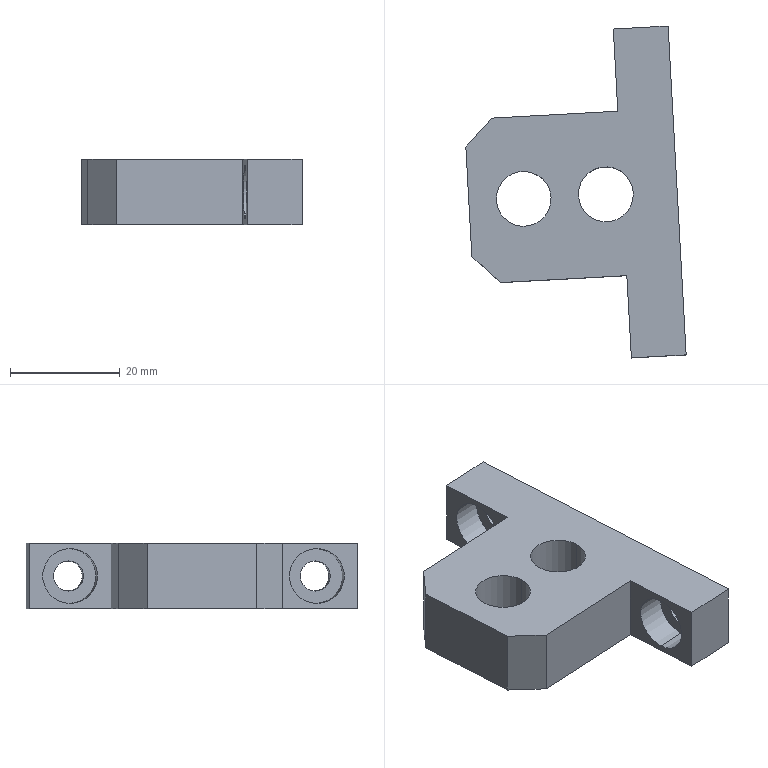Component | SolidWorks | BearingPressPartK-1 | 1 solid | 26 faces | box 40.13 x 60.46 x 12 mm | volume 14028 mm3 | plane 14 | cylinder 12 | commonest cylinder face diameters 10 x8 5.5 x4
build123d program:
from build123d import *

# Parameters (mm, degrees)
SKETCH1_W                                       = 38
SKETCH1_H                                       = 30
BOSS_EXTRUDE1_DEPTH                             = 12
M10X1_25_TAPPED_HOLE1_D                         = 10
M10X1_25_TAPPED_HOLE1_DEPTH                     = 23.75
M10X1_25_TAPPED_HOLE1_TIP                       = 3.004
CHAMFER1_SIZE                                   = 5
SKETCH6_W                                       = 10
SKETCH6_H                                       = 12
BOSS_EXTRUDE2_DEPTH                             = 15
SKETCH7_W                                       = 10
SKETCH7_H                                       = 12
BOSS_EXTRUDE3_DEPTH                             = 15
M5_HEX_SOCKET_HEAD_CAP_SCREW_CBORE1_D           = 5.5
M5_HEX_SOCKET_HEAD_CAP_SCREW_CBORE1_CBORE_D     = 10
M5_HEX_SOCKET_HEAD_CAP_SCREW_CBORE1_CBORE_DEPTH = 5.4


with BuildPart() as part:
    # Sketch1 → Boss-Extrude1 (new body)
    with BuildSketch(Plane.XY):
        with Locations((19, 15)):
            Rectangle(SKETCH1_W, SKETCH1_H)
    extrude(amount=BOSS_EXTRUDE1_DEPTH)

    # M10x1.25 Tapped Hole1
    with Locations(Plane.XY.offset(12)):
        with Locations((25, 15), (10, 15)):
            Hole(M10X1_25_TAPPED_HOLE1_D / 2, depth=M10X1_25_TAPPED_HOLE1_DEPTH)
            with Locations((0, 0, -(M10X1_25_TAPPED_HOLE1_DEPTH + M10X1_25_TAPPED_HOLE1_TIP / 2))):  # 118° drill point
                Cone(0, M10X1_25_TAPPED_HOLE1_D / 2, M10X1_25_TAPPED_HOLE1_TIP, mode=Mode.SUBTRACT)

    # Chamfer1
    chamfer1_edges = [part.edges().sort_by_distance(p)[0] for p in [
        (0, 30, 6),
        (0, 0, 6),
    ]]
    chamfer(chamfer1_edges, length=CHAMFER1_SIZE)

    # Sketch6 → Boss-Extrude2 (add)
    with BuildSketch(Plane.XZ):
        with Locations((33, 6)):
            Rectangle(SKETCH6_W, SKETCH6_H)
    extrude(amount=BOSS_EXTRUDE2_DEPTH)

    # Sketch7 → Boss-Extrude3 (add)
    with BuildSketch(Plane(origin=(0, 30, 0), x_dir=(1, 0, 0), z_dir=(0, 1, 0))):
        with Locations((33, -6)):
            Rectangle(SKETCH7_W, SKETCH7_H)
    extrude(amount=BOSS_EXTRUDE3_DEPTH)

    # M5 Hex Socket Head Cap Screw CBORE1 (through all)
    with Locations(Plane.ZY.offset(-28)):
        with Locations((6, -7.5), (6, 37.5)):
            CounterBoreHole(M5_HEX_SOCKET_HEAD_CAP_SCREW_CBORE1_D / 2, M5_HEX_SOCKET_HEAD_CAP_SCREW_CBORE1_CBORE_D / 2, M5_HEX_SOCKET_HEAD_CAP_SCREW_CBORE1_CBORE_DEPTH)


solid = part.part

# Placed as in the assembly
solid = solid.moved(Location((348.421, 102.495, -236.818), (0, 0, 3.137)))
STEP:
#1=CARTESIAN_POINT('',(15.047,3.812,-9.284));
#2=VERTEX_POINT('',#1);
#3=CARTESIAN_POINT('',(15.047,3.812,-8.89));
#4=VERTEX_POINT('',#3);
#5=CARTESIAN_POINT('',(15.047,3.812,-9.087));
#6=DIRECTION('',(-0.9985,-0.05472,0.));
#7=DIRECTION('',(0.,0.,1.));
#8=AXIS2_PLACEMENT_3D('',#5,#6,#7);
#9=CIRCLE('',#8,0.1969);
#10=EDGE_CURVE('',#2,#4,#9,.T.);
#11=ORIENTED_EDGE('',*,*,#10,.F.);
#12=CARTESIAN_POINT('',(14.834,3.801,-9.284));
#13=VERTEX_POINT('',#12);
#14=CARTESIAN_POINT('',(14.834,3.801,-9.284));
#15=DIRECTION('',(-0.9985,-0.05472,0.));
#16=VECTOR('',#15,39.37);
#17=LINE('',#14,#16);
#18=EDGE_CURVE('',#2,#13,#17,.T.);
#19=ORIENTED_EDGE('',*,*,#18,.T.);
#20=CARTESIAN_POINT('',(14.834,3.801,-8.89));
#21=VERTEX_POINT('',#20);
#22=CARTESIAN_POINT('',(14.834,3.801,-9.087));
#23=DIRECTION('',(-0.9985,-0.05472,0.));
#24=DIRECTION('',(0.,0.,1.));
#25=AXIS2_PLACEMENT_3D('',#22,#23,#24);
#26=CIRCLE('',#25,0.1969);
#27=EDGE_CURVE('',#13,#21,#26,.T.);
#28=ORIENTED_EDGE('',*,*,#27,.T.);
#29=CARTESIAN_POINT('',(14.834,3.801,-8.89));
#30=DIRECTION('',(-0.9985,-0.05472,0.));
#31=VECTOR('',#30,39.37);
#32=LINE('',#29,#31);
#33=EDGE_CURVE('',#4,#21,#32,.T.);
#34=ORIENTED_EDGE('',*,*,#33,.F.);
#35=EDGE_LOOP('',(#11,#19,#28,#34));
#36=FACE_OUTER_BOUND('',#35,.T.);
#37=CARTESIAN_POINT('',(14.834,3.801,-9.087));
#38=DIRECTION('',(-0.9985,-0.05472,0.));
#39=DIRECTION('',(0.,0.,1.));
#40=AXIS2_PLACEMENT_3D('',#37,#38,#39);
#41=CYLINDRICAL_SURFACE('',#40,0.1969);
#42=ADVANCED_FACE('',(#36),#41,.F.);
#43=CARTESIAN_POINT('',(15.227,3.822,-9.196));
#44=VERTEX_POINT('',#43);
#45=CARTESIAN_POINT('',(15.227,3.822,-8.979));
#46=VERTEX_POINT('',#45);
#47=CARTESIAN_POINT('',(15.227,3.822,-9.087));
#48=DIRECTION('',(-0.9985,-0.05472,0.));
#49=DIRECTION('',(0.,0.,1.));
#50=AXIS2_PLACEMENT_3D('',#47,#48,#49);
#51=CIRCLE('',#50,0.1083);
#52=EDGE_CURVE('',#44,#46,#51,.T.);
#53=ORIENTED_EDGE('',*,*,#52,.F.);
#54=CARTESIAN_POINT('',(15.047,3.812,-9.196));
#55=VERTEX_POINT('',#54);
#56=CARTESIAN_POINT('',(14.834,3.801,-9.196));
#57=DIRECTION('',(-0.9985,-0.05472,0.));
#58=VECTOR('',#57,39.37);
#59=LINE('',#56,#58);
#60=EDGE_CURVE('',#44,#55,#59,.T.);
#61=ORIENTED_EDGE('',*,*,#60,.T.);
#62=CARTESIAN_POINT('',(15.047,3.812,-8.979));
#63=VERTEX_POINT('',#62);
#64=CARTESIAN_POINT('',(15.047,3.812,-9.087));
#65=DIRECTION('',(-0.9985,-0.05472,0.));
#66=DIRECTION('',(0.,0.,1.));
#67=AXIS2_PLACEMENT_3D('',#64,#65,#66);
#68=CIRCLE('',#67,0.1083);
#69=EDGE_CURVE('',#55,#63,#68,.T.);
#70=ORIENTED_EDGE('',*,*,#69,.T.);
#71=CARTESIAN_POINT('',(14.834,3.801,-8.979));
#72=DIRECTION('',(-0.9985,-0.05472,0.));
#73=VECTOR('',#72,39.37);
#74=LINE('',#71,#73);
#75=EDGE_CURVE('',#46,#63,#74,.T.);
#76=ORIENTED_EDGE('',*,*,#75,.F.);
#77=EDGE_LOOP('',(#53,#61,#70,#76));
#78=FACE_OUTER_BOUND('',#77,.T.);
#79=CARTESIAN_POINT('',(14.834,3.801,-9.087));
#80=DIRECTION('',(-0.9985,-0.05472,0.));
#81=DIRECTION('',(0.,0.,1.));
#82=AXIS2_PLACEMENT_3D('',#79,#80,#81);
#83=CYLINDRICAL_SURFACE('',#82,0.1083);
#84=ADVANCED_FACE('',(#78),#83,.F.);
#85=CARTESIAN_POINT('',(14.95,5.581,-9.284));
#86=VERTEX_POINT('',#85);
#87=CARTESIAN_POINT('',(14.95,5.581,-8.89));
#88=VERTEX_POINT('',#87);
#89=CARTESIAN_POINT('',(14.95,5.581,-9.087));
#90=DIRECTION('',(-0.9985,-0.05472,0.));
#91=DIRECTION('',(0.,0.,1.));
#92=AXIS2_PLACEMENT_3D('',#89,#90,#91);
#93=CIRCLE('',#92,0.1969);
#94=EDGE_CURVE('',#86,#88,#93,.T.);
#95=ORIENTED_EDGE('',*,*,#94,.F.);
#96=CARTESIAN_POINT('',(14.737,5.57,-9.284));
#97=VERTEX_POINT('',#96);
#98=CARTESIAN_POINT('',(14.737,5.57,-9.284));
#99=DIRECTION('',(-0.9985,-0.05472,0.));
#100=VECTOR('',#99,39.37);
#101=LINE('',#98,#100);
#102=EDGE_CURVE('',#86,#97,#101,.T.);
#103=ORIENTED_EDGE('',*,*,#102,.T.);
#104=CARTESIAN_POINT('',(14.737,5.57,-8.89));
#105=VERTEX_POINT('',#104);
#106=CARTESIAN_POINT('',(14.737,5.57,-9.087));
#107=DIRECTION('',(-0.9985,-0.05472,0.));
#108=DIRECTION('',(0.,0.,1.));
#109=AXIS2_PLACEMENT_3D('',#106,#107,#108);
#110=CIRCLE('',#109,0.1969);
#111=EDGE_CURVE('',#97,#105,#110,.T.);
#112=ORIENTED_EDGE('',*,*,#111,.T.);
#113=CARTESIAN_POINT('',(14.737,5.57,-8.89));
#114=DIRECTION('',(-0.9985,-0.05472,0.));
#115=VECTOR('',#114,39.37);
#116=LINE('',#113,#115);
#117=EDGE_CURVE('',#88,#105,#116,.T.);
#118=ORIENTED_EDGE('',*,*,#117,.F.);
#119=EDGE_LOOP('',(#95,#103,#112,#118));
#120=FACE_OUTER_BOUND('',#119,.T.);
#121=CARTESIAN_POINT('',(14.737,5.57,-9.087));
#122=DIRECTION('',(-0.9985,-0.05472,0.));
#123=DIRECTION('',(0.,0.,1.));
#124=AXIS2_PLACEMENT_3D('',#121,#122,#123);
#125=CYLINDRICAL_SURFACE('',#124,0.1969);
#126=ADVANCED_FACE('',(#120),#125,.F.);
#127=CARTESIAN_POINT('',(15.13,5.591,-9.196));
#128=VERTEX_POINT('',#127);
#129=CARTESIAN_POINT('',(15.13,5.591,-8.979));
#130=VERTEX_POINT('',#129);
#131=CARTESIAN_POINT('',(15.13,5.591,-9.087));
#132=DIRECTION('',(-0.9985,-0.05472,0.));
#133=DIRECTION('',(0.,0.,1.));
#134=AXIS2_PLACEMENT_3D('',#131,#132,#133);
#135=CIRCLE('',#134,0.1083);
#136=EDGE_CURVE('',#128,#130,#135,.T.);
#137=ORIENTED_EDGE('',*,*,#136,.F.);
#138=CARTESIAN_POINT('',(14.95,5.581,-9.196));
#139=VERTEX_POINT('',#138);
#140=CARTESIAN_POINT('',(14.737,5.57,-9.196));
#141=DIRECTION('',(-0.9985,-0.05472,0.));
#142=VECTOR('',#141,39.37);
#143=LINE('',#140,#142);
#144=EDGE_CURVE('',#128,#139,#143,.T.);
#145=ORIENTED_EDGE('',*,*,#144,.T.);
#146=CARTESIAN_POINT('',(14.95,5.581,-8.979));
#147=VERTEX_POINT('',#146);
#148=CARTESIAN_POINT('',(14.95,5.581,-9.087));
#149=DIRECTION('',(-0.9985,-0.05472,0.));
#150=DIRECTION('',(0.,0.,1.));
#151=AXIS2_PLACEMENT_3D('',#148,#149,#150);
#152=CIRCLE('',#151,0.1083);
#153=EDGE_CURVE('',#139,#147,#152,.T.);
#154=ORIENTED_EDGE('',*,*,#153,.T.);
#155=CARTESIAN_POINT('',(14.737,5.57,-8.979));
#156=DIRECTION('',(-0.9985,-0.05472,0.));
#157=VECTOR('',#156,39.37);
#158=LINE('',#155,#157);
#159=EDGE_CURVE('',#130,#147,#158,.T.);
#160=ORIENTED_EDGE('',*,*,#159,.F.);
#161=EDGE_LOOP('',(#137,#145,#154,#160));
#162=FACE_OUTER_BOUND('',#161,.T.);
#163=CARTESIAN_POINT('',(14.737,5.57,-9.087));
#164=DIRECTION('',(-0.9985,-0.05472,0.));
#165=DIRECTION('',(0.,0.,1.));
#166=AXIS2_PLACEMENT_3D('',#163,#164,#165);
#167=CYLINDRICAL_SURFACE('',#166,0.1083);
#168=ADVANCED_FACE('',(#162),#167,.F.);
#169=CARTESIAN_POINT('',(14.864,4.69,-9.324));
#170=VERTEX_POINT('',#169);
#171=CARTESIAN_POINT('',(14.471,4.668,-9.324));
#172=VERTEX_POINT('',#171);
#173=CARTESIAN_POINT('',(14.668,4.679,-9.324));
#174=DIRECTION('',(-0.,-0.,-1.));
#175=DIRECTION('',(-0.9985,-0.05472,0.));
#176=AXIS2_PLACEMENT_3D('',#173,#174,#175);
#177=CIRCLE('',#176,0.1969);
#178=EDGE_CURVE('',#170,#172,#177,.T.);
#179=ORIENTED_EDGE('',*,*,#178,.T.);
#180=CARTESIAN_POINT('',(14.471,4.668,-8.851));
#181=VERTEX_POINT('',#180);
#182=CARTESIAN_POINT('',(14.471,4.668,-8.851));
#183=DIRECTION('',(0.,0.,1.));
#184=VECTOR('',#183,39.37);
#185=LINE('',#182,#184);
#186=EDGE_CURVE('',#172,#181,#185,.T.);
#187=ORIENTED_EDGE('',*,*,#186,.T.);
#188=CARTESIAN_POINT('',(14.864,4.69,-8.851));
#189=VERTEX_POINT('',#188);
#190=CARTESIAN_POINT('',(14.668,4.679,-8.851));
#191=DIRECTION('',(0.,0.,1.));
#192=DIRECTION('',(0.9985,0.05472,0.));
#193=AXIS2_PLACEMENT_3D('',#190,#191,#192);
#194=CIRCLE('',#193,0.1969);
#195=EDGE_CURVE('',#181,#189,#194,.T.);
#196=ORIENTED_EDGE('',*,*,#195,.T.);
#197=CARTESIAN_POINT('',(14.864,4.69,-8.851));
#198=DIRECTION('',(0.,0.,1.));
#199=VECTOR('',#198,39.37);
#200=LINE('',#197,#199);
#201=EDGE_CURVE('',#170,#189,#200,.T.);
#202=ORIENTED_EDGE('',*,*,#201,.F.);
#203=EDGE_LOOP('',(#179,#187,#196,#202));
#204=FACE_OUTER_BOUND('',#203,.T.);
#205=CARTESIAN_POINT('',(14.668,4.679,-8.851));
#206=DIRECTION('',(0.,0.,1.));
#207=DIRECTION('',(0.9985,0.05472,0.));
#208=AXIS2_PLACEMENT_3D('',#205,#206,#207);
#209=CYLINDRICAL_SURFACE('',#208,0.1969);
#210=ADVANCED_FACE('',(#204),#209,.F.);
#211=CARTESIAN_POINT('',(14.275,4.657,-9.324));
#212=VERTEX_POINT('',#211);
#213=CARTESIAN_POINT('',(13.882,4.636,-9.324));
#214=VERTEX_POINT('',#213);
#215=CARTESIAN_POINT('',(14.078,4.646,-9.324));
#216=DIRECTION('',(-0.,-0.,-1.));
#217=DIRECTION('',(-0.9985,-0.05472,0.));
#218=AXIS2_PLACEMENT_3D('',#215,#216,#217);
#219=CIRCLE('',#218,0.1969);
#220=EDGE_CURVE('',#212,#214,#219,.T.);
#221=ORIENTED_EDGE('',*,*,#220,.T.);
#222=CARTESIAN_POINT('',(13.882,4.636,-8.851));
#223=VERTEX_POINT('',#222);
#224=CARTESIAN_POINT('',(13.882,4.636,-8.851));
#225=DIRECTION('',(0.,0.,1.));
#226=VECTOR('',#225,39.37);
#227=LINE('',#224,#226);
#228=EDGE_CURVE('',#214,#223,#227,.T.);
#229=ORIENTED_EDGE('',*,*,#228,.T.);
#230=CARTESIAN_POINT('',(14.275,4.657,-8.851));
#231=VERTEX_POINT('',#230);
#232=CARTESIAN_POINT('',(14.078,4.646,-8.851));
#233=DIRECTION('',(0.,0.,1.));
#234=DIRECTION('',(0.9985,0.05472,0.));
#235=AXIS2_PLACEMENT_3D('',#232,#233,#234);
#236=CIRCLE('',#235,0.1969);
#237=EDGE_CURVE('',#223,#231,#236,.T.);
#238=ORIENTED_EDGE('',*,*,#237,.T.);
#239=CARTESIAN_POINT('',(14.275,4.657,-8.851));
#240=DIRECTION('',(0.,0.,1.));
#241=VECTOR('',#240,39.37);
#242=LINE('',#239,#241);
#243=EDGE_CURVE('',#212,#231,#242,.T.);
#244=ORIENTED_EDGE('',*,*,#243,.F.);
#245=EDGE_LOOP('',(#221,#229,#238,#244));
#246=FACE_OUTER_BOUND('',#245,.T.);
#247=CARTESIAN_POINT('',(14.078,4.646,-8.851));
#248=DIRECTION('',(0.,0.,1.));
#249=DIRECTION('',(0.9985,0.05472,0.));
#250=AXIS2_PLACEMENT_3D('',#247,#248,#249);
#251=CYLINDRICAL_SURFACE('',#250,0.1969);
#252=ADVANCED_FACE('',(#246),#251,.F.);
#253=CARTESIAN_POINT('',(14.753,5.275,-9.324));
#254=VERTEX_POINT('',#253);
#255=CARTESIAN_POINT('',(14.753,5.275,-8.851));
#256=VERTEX_POINT('',#255);
#257=CARTESIAN_POINT('',(14.753,5.275,-9.324));
#258=DIRECTION('',(0.,0.,1.));
#259=VECTOR('',#258,39.37);
#260=LINE('',#257,#259);
#261=EDGE_CURVE('',#254,#256,#260,.T.);
#262=ORIENTED_EDGE('',*,*,#261,.F.);
#263=CARTESIAN_POINT('',(13.849,5.225,-9.324));
#264=VERTEX_POINT('',#263);
#265=CARTESIAN_POINT('',(13.653,5.215,-9.324));
#266=DIRECTION('',(-0.9985,-0.05472,0.));
#267=VECTOR('',#266,39.37);
#268=LINE('',#265,#267);
#269=EDGE_CURVE('',#254,#264,#268,.T.);
#270=ORIENTED_EDGE('',*,*,#269,.T.);
#271=CARTESIAN_POINT('',(13.849,5.225,-8.851));
#272=VERTEX_POINT('',#271);
#273=CARTESIAN_POINT('',(13.849,5.225,-8.851));
#274=DIRECTION('',(0.,0.,1.));
#275=VECTOR('',#274,39.37);
#276=LINE('',#273,#275);
#277=EDGE_CURVE('',#264,#272,#276,.T.);
#278=ORIENTED_EDGE('',*,*,#277,.T.);
#279=CARTESIAN_POINT('',(13.653,5.215,-8.851));
#280=DIRECTION('',(-0.9985,-0.05472,0.));
#281=VECTOR('',#280,39.37);
#282=LINE('',#279,#281);
#283=EDGE_CURVE('',#256,#272,#282,.T.);
#284=ORIENTED_EDGE('',*,*,#283,.F.);
#285=EDGE_LOOP('',(#262,#270,#278,#284));
#286=FACE_OUTER_BOUND('',#285,.T.);
#287=CARTESIAN_POINT('',(13.653,5.215,-8.851));
#288=DIRECTION('',(0.05472,-0.9985,0.));
#289=DIRECTION('',(-0.,-0.,-1.));
#290=AXIS2_PLACEMENT_3D('',#287,#288,#289);
#291=PLANE('',#290);
#292=ADVANCED_FACE('',(#286),#291,.F.);
#293=CARTESIAN_POINT('',(14.818,4.096,-8.851));
#294=VERTEX_POINT('',#293);
#295=CARTESIAN_POINT('',(14.818,4.096,-9.324));
#296=VERTEX_POINT('',#295);
#297=CARTESIAN_POINT('',(14.818,4.096,-8.851));
#298=DIRECTION('',(-0.,-0.,-1.));
#299=VECTOR('',#298,39.37);
#300=LINE('',#297,#299);
#301=EDGE_CURVE('',#294,#296,#300,.T.);
#302=ORIENTED_EDGE('',*,*,#301,.F.);
#303=CARTESIAN_POINT('',(13.914,4.046,-8.851));
#304=VERTEX_POINT('',#303);
#305=CARTESIAN_POINT('',(13.717,4.035,-8.851));
#306=DIRECTION('',(0.9985,0.05472,-0.));
#307=VECTOR('',#306,39.37);
#308=LINE('',#305,#307);
#309=EDGE_CURVE('',#304,#294,#308,.T.);
#310=ORIENTED_EDGE('',*,*,#309,.F.);
#311=CARTESIAN_POINT('',(13.914,4.046,-9.324));
#312=VERTEX_POINT('',#311);
#313=CARTESIAN_POINT('',(13.914,4.046,-8.851));
#314=DIRECTION('',(-0.,-0.,-1.));
#315=VECTOR('',#314,39.37);
#316=LINE('',#313,#315);
#317=EDGE_CURVE('',#304,#312,#316,.T.);
#318=ORIENTED_EDGE('',*,*,#317,.T.);
#319=CARTESIAN_POINT('',(13.717,4.035,-9.324));
#320=DIRECTION('',(0.9985,0.05472,-0.));
#321=VECTOR('',#320,39.37);
#322=LINE('',#319,#321);
#323=EDGE_CURVE('',#312,#296,#322,.T.);
#324=ORIENTED_EDGE('',*,*,#323,.T.);
#325=EDGE_LOOP('',(#302,#310,#318,#324));
#326=FACE_OUTER_BOUND('',#325,.T.);
#327=CARTESIAN_POINT('',(13.717,4.035,-8.851));
#328=DIRECTION('',(-0.05472,0.9985,-0.));
#329=DIRECTION('',(0.,0.,1.));
#330=AXIS2_PLACEMENT_3D('',#327,#328,#329);
#331=PLANE('',#330);
#332=ADVANCED_FACE('',(#326),#331,.F.);
#333=CARTESIAN_POINT('',(14.078,4.646,-8.851));
#334=DIRECTION('',(0.,0.,1.));
#335=DIRECTION('',(0.9985,0.05472,0.));
#336=AXIS2_PLACEMENT_3D('',#333,#334,#335);
#337=CIRCLE('',#336,0.1969);
#338=EDGE_CURVE('',#231,#223,#337,.T.);
#339=ORIENTED_EDGE('',*,*,#338,.F.);
#340=ORIENTED_EDGE('',*,*,#237,.F.);
#341=EDGE_LOOP('',(#339,#340));
#342=FACE_BOUND('',#341,.T.);
#343=CARTESIAN_POINT('',(13.664,5.018,-8.851));
#344=VERTEX_POINT('',#343);
#345=CARTESIAN_POINT('',(13.707,4.232,-8.851));
#346=VERTEX_POINT('',#345);
#347=CARTESIAN_POINT('',(13.717,4.035,-8.851));
#348=DIRECTION('',(0.05472,-0.9985,0.));
#349=VECTOR('',#348,39.37);
#350=LINE('',#347,#349);
#351=EDGE_CURVE('',#344,#346,#350,.T.);
#352=ORIENTED_EDGE('',*,*,#351,.T.);
#353=CARTESIAN_POINT('',(13.914,4.046,-8.851));
#354=DIRECTION('',(0.7447,-0.6674,0.));
#355=VECTOR('',#354,39.37);
#356=LINE('',#353,#355);
#357=EDGE_CURVE('',#346,#304,#356,.T.);
#358=ORIENTED_EDGE('',*,*,#357,.T.);
#359=ORIENTED_EDGE('',*,*,#309,.T.);
#360=CARTESIAN_POINT('',(14.85,3.506,-8.851));
#361=VERTEX_POINT('',#360);
#362=CARTESIAN_POINT('',(14.85,3.506,-8.851));
#363=DIRECTION('',(-0.05472,0.9985,-0.));
#364=VECTOR('',#363,39.37);
#365=LINE('',#362,#364);
#366=EDGE_CURVE('',#361,#294,#365,.T.);
#367=ORIENTED_EDGE('',*,*,#366,.F.);
#368=CARTESIAN_POINT('',(15.244,3.527,-8.851));
#369=VERTEX_POINT('',#368);
#370=CARTESIAN_POINT('',(15.244,3.527,-8.851));
#371=DIRECTION('',(-0.9985,-0.05472,-0.));
#372=VECTOR('',#371,39.37);
#373=LINE('',#370,#372);
#374=EDGE_CURVE('',#369,#361,#373,.T.);
#375=ORIENTED_EDGE('',*,*,#374,.F.);
#376=CARTESIAN_POINT('',(15.114,5.886,-8.851));
#377=VERTEX_POINT('',#376);
#378=CARTESIAN_POINT('',(15.211,4.117,-8.851));
#379=DIRECTION('',(-0.05472,0.9985,-0.));
#380=VECTOR('',#379,39.37);
#381=LINE('',#378,#380);
#382=EDGE_CURVE('',#369,#377,#381,.T.);
#383=ORIENTED_EDGE('',*,*,#382,.T.);
#384=CARTESIAN_POINT('',(14.721,5.865,-8.851));
#385=VERTEX_POINT('',#384);
#386=CARTESIAN_POINT('',(15.114,5.886,-8.851));
#387=DIRECTION('',(0.9985,0.05472,-0.));
#388=VECTOR('',#387,39.37);
#389=LINE('',#386,#388);
#390=EDGE_CURVE('',#385,#377,#389,.T.);
#391=ORIENTED_EDGE('',*,*,#390,.F.);
#392=CARTESIAN_POINT('',(14.721,5.865,-8.851));
#393=DIRECTION('',(0.05472,-0.9985,0.));
#394=VECTOR('',#393,39.37);
#395=LINE('',#392,#394);
#396=EDGE_CURVE('',#385,#256,#395,.T.);
#397=ORIENTED_EDGE('',*,*,#396,.T.);
#398=ORIENTED_EDGE('',*,*,#283,.T.);
#399=CARTESIAN_POINT('',(13.664,5.018,-8.851));
#400=DIRECTION('',(-0.6674,-0.7447,0.));
#401=VECTOR('',#400,39.37);
#402=LINE('',#399,#401);
#403=EDGE_CURVE('',#272,#344,#402,.T.);
#404=ORIENTED_EDGE('',*,*,#403,.T.);
#405=EDGE_LOOP('',(#352,#358,#359,#367,#375,#383,#391,#397,#398,#404));
#406=FACE_OUTER_BOUND('',#405,.T.);
#407=CARTESIAN_POINT('',(14.668,4.679,-8.851));
#408=DIRECTION('',(0.,0.,1.));
#409=DIRECTION('',(0.9985,0.05472,0.));
#410=AXIS2_PLACEMENT_3D('',#407,#408,#409);
#411=CIRCLE('',#410,0.1969);
#412=EDGE_CURVE('',#189,#181,#411,.T.);
#413=ORIENTED_EDGE('',*,*,#412,.F.);
#414=ORIENTED_EDGE('',*,*,#195,.F.);
#415=EDGE_LOOP('',(#413,#414));
#416=FACE_BOUND('',#415,.T.);
#417=CARTESIAN_POINT('',(13.717,4.035,-8.851));
#418=DIRECTION('',(-0.,-0.,-1.));
#419=DIRECTION('',(-0.9985,-0.05472,0.));
#420=AXIS2_PLACEMENT_3D('',#417,#418,#419);
#421=PLANE('',#420);
#422=ADVANCED_FACE('',(#342,#406,#416),#421,.F.);
#423=CARTESIAN_POINT('',(13.664,5.018,-9.324));
#424=VERTEX_POINT('',#423);
#425=CARTESIAN_POINT('',(13.707,4.232,-9.324));
#426=VERTEX_POINT('',#425);
#427=CARTESIAN_POINT('',(13.717,4.035,-9.324));
#428=DIRECTION('',(0.05472,-0.9985,0.));
#429=VECTOR('',#428,39.37);
#430=LINE('',#427,#429);
#431=EDGE_CURVE('',#424,#426,#430,.T.);
#432=ORIENTED_EDGE('',*,*,#431,.T.);
#433=CARTESIAN_POINT('',(13.707,4.232,-8.851));
#434=DIRECTION('',(0.,0.,1.));
#435=VECTOR('',#434,39.37);
#436=LINE('',#433,#435);
#437=EDGE_CURVE('',#426,#346,#436,.T.);
#438=ORIENTED_EDGE('',*,*,#437,.T.);
#439=ORIENTED_EDGE('',*,*,#351,.F.);
#440=CARTESIAN_POINT('',(13.664,5.018,-8.851));
#441=DIRECTION('',(-0.,-0.,-1.));
#442=VECTOR('',#441,39.37);
#443=LINE('',#440,#442);
#444=EDGE_CURVE('',#344,#424,#443,.T.);
#445=ORIENTED_EDGE('',*,*,#444,.T.);
#446=EDGE_LOOP('',(#432,#438,#439,#445));
#447=FACE_OUTER_BOUND('',#446,.T.);
#448=CARTESIAN_POINT('',(13.717,4.035,-8.851));
#449=DIRECTION('',(0.9985,0.05472,-0.));
#450=DIRECTION('',(-0.,-0.,-1.));
#451=AXIS2_PLACEMENT_3D('',#448,#449,#450);
#452=PLANE('',#451);
#453=ADVANCED_FACE('',(#447),#452,.F.);
#454=CARTESIAN_POINT('',(15.227,3.822,-9.087));
#455=DIRECTION('',(-0.9985,-0.05472,0.));
#456=DIRECTION('',(0.,0.,1.));
#457=AXIS2_PLACEMENT_3D('',#454,#455,#456);
#458=CIRCLE('',#457,0.1083);
#459=EDGE_CURVE('',#46,#44,#458,.T.);
#460=ORIENTED_EDGE('',*,*,#459,.T.);
#461=ORIENTED_EDGE('',*,*,#52,.T.);
#462=EDGE_LOOP('',(#460,#461));
#463=FACE_BOUND('',#462,.T.);
#464=CARTESIAN_POINT('',(15.13,5.591,-9.087));
#465=DIRECTION('',(-0.9985,-0.05472,0.));
#466=DIRECTION('',(0.,0.,1.));
#467=AXIS2_PLACEMENT_3D('',#464,#465,#466);
#468=CIRCLE('',#467,0.1083);
#469=EDGE_CURVE('',#130,#128,#468,.T.);
#470=ORIENTED_EDGE('',*,*,#469,.T.);
#471=ORIENTED_EDGE('',*,*,#136,.T.);
#472=EDGE_LOOP('',(#470,#471));
#473=FACE_BOUND('',#472,.T.);
#474=CARTESIAN_POINT('',(15.244,3.527,-9.324));
#475=VERTEX_POINT('',#474);
#476=CARTESIAN_POINT('',(15.114,5.886,-9.324));
#477=VERTEX_POINT('',#476);
#478=CARTESIAN_POINT('',(15.211,4.117,-9.324));
#479=DIRECTION('',(-0.05472,0.9985,-0.));
#480=VECTOR('',#479,39.37);
#481=LINE('',#478,#480);
#482=EDGE_CURVE('',#475,#477,#481,.T.);
#483=ORIENTED_EDGE('',*,*,#482,.T.);
#484=CARTESIAN_POINT('',(15.114,5.886,-9.324));
#485=DIRECTION('',(-0.,-0.,-1.));
#486=VECTOR('',#485,39.37);
#487=LINE('',#484,#486);
#488=EDGE_CURVE('',#377,#477,#487,.T.);
#489=ORIENTED_EDGE('',*,*,#488,.F.);
#490=ORIENTED_EDGE('',*,*,#382,.F.);
#491=CARTESIAN_POINT('',(15.244,3.527,-8.851));
#492=DIRECTION('',(0.,0.,1.));
#493=VECTOR('',#492,39.37);
#494=LINE('',#491,#493);
#495=EDGE_CURVE('',#475,#369,#494,.T.);
#496=ORIENTED_EDGE('',*,*,#495,.F.);
#497=EDGE_LOOP('',(#483,#489,#490,#496));
#498=FACE_OUTER_BOUND('',#497,.T.);
#499=CARTESIAN_POINT('',(15.211,4.117,-8.851));
#500=DIRECTION('',(-0.9985,-0.05472,0.));
#501=DIRECTION('',(0.,0.,1.));
#502=AXIS2_PLACEMENT_3D('',#499,#500,#501);
#503=PLANE('',#502);
#504=ADVANCED_FACE('',(#463,#473,#498),#503,.F.);
#505=ORIENTED_EDGE('',*,*,#178,.F.);
#506=CARTESIAN_POINT('',(14.668,4.679,-9.324));
#507=DIRECTION('',(-0.,-0.,-1.));
#508=DIRECTION('',(-0.9985,-0.05472,0.));
#509=AXIS2_PLACEMENT_3D('',#506,#507,#508);
#510=CIRCLE('',#509,0.1969);
#511=EDGE_CURVE('',#172,#170,#510,.T.);
#512=ORIENTED_EDGE('',*,*,#511,.F.);
#513=EDGE_LOOP('',(#505,#512));
#514=FACE_BOUND('',#513,.T.);
#515=ORIENTED_EDGE('',*,*,#220,.F.);
#516=CARTESIAN_POINT('',(14.078,4.646,-9.324));
#517=DIRECTION('',(-0.,-0.,-1.));
#518=DIRECTION('',(-0.9985,-0.05472,0.));
#519=AXIS2_PLACEMENT_3D('',#516,#517,#518);
#520=CIRCLE('',#519,0.1969);
#521=EDGE_CURVE('',#214,#212,#520,.T.);
#522=ORIENTED_EDGE('',*,*,#521,.F.);
#523=EDGE_LOOP('',(#515,#522));
#524=FACE_BOUND('',#523,.T.);
#525=ORIENTED_EDGE('',*,*,#323,.F.);
#526=CARTESIAN_POINT('',(13.81,4.139,-9.324));
#527=DIRECTION('',(-0.7447,0.6674,-0.));
#528=VECTOR('',#527,39.37);
#529=LINE('',#526,#528);
#530=EDGE_CURVE('',#312,#426,#529,.T.);
#531=ORIENTED_EDGE('',*,*,#530,.T.);
#532=ORIENTED_EDGE('',*,*,#431,.F.);
#533=CARTESIAN_POINT('',(13.199,4.5,-9.324));
#534=DIRECTION('',(0.6674,0.7447,-0.));
#535=VECTOR('',#534,39.37);
#536=LINE('',#533,#535);
#537=EDGE_CURVE('',#424,#264,#536,.T.);
#538=ORIENTED_EDGE('',*,*,#537,.T.);
#539=ORIENTED_EDGE('',*,*,#269,.F.);
#540=CARTESIAN_POINT('',(14.721,5.865,-9.324));
#541=VERTEX_POINT('',#540);
#542=CARTESIAN_POINT('',(14.721,5.865,-9.324));
#543=DIRECTION('',(0.05472,-0.9985,0.));
#544=VECTOR('',#543,39.37);
#545=LINE('',#542,#544);
#546=EDGE_CURVE('',#541,#254,#545,.T.);
#547=ORIENTED_EDGE('',*,*,#546,.F.);
#548=CARTESIAN_POINT('',(15.114,5.886,-9.324));
#549=DIRECTION('',(-0.9985,-0.05472,0.));
#550=VECTOR('',#549,39.37);
#551=LINE('',#548,#550);
#552=EDGE_CURVE('',#477,#541,#551,.T.);
#553=ORIENTED_EDGE('',*,*,#552,.F.);
#554=ORIENTED_EDGE('',*,*,#482,.F.);
#555=CARTESIAN_POINT('',(14.85,3.506,-9.324));
#556=VERTEX_POINT('',#555);
#557=CARTESIAN_POINT('',(15.244,3.527,-9.324));
#558=DIRECTION('',(0.9985,0.05472,-0.));
#559=VECTOR('',#558,39.37);
#560=LINE('',#557,#559);
#561=EDGE_CURVE('',#556,#475,#560,.T.);
#562=ORIENTED_EDGE('',*,*,#561,.F.);
#563=CARTESIAN_POINT('',(14.85,3.506,-9.324));
#564=DIRECTION('',(-0.05472,0.9985,-0.));
#565=VECTOR('',#564,39.37);
#566=LINE('',#563,#565);
#567=EDGE_CURVE('',#556,#296,#566,.T.);
#568=ORIENTED_EDGE('',*,*,#567,.T.);
#569=EDGE_LOOP('',(#525,#531,#532,#538,#539,#547,#553,#554,#562,#568));
#570=FACE_OUTER_BOUND('',#569,.T.);
#571=CARTESIAN_POINT('',(13.717,4.035,-9.324));
#572=DIRECTION('',(-0.,-0.,-1.));
#573=DIRECTION('',(-0.9985,-0.05472,0.));
#574=AXIS2_PLACEMENT_3D('',#571,#572,#573);
#575=PLANE('',#574);
#576=ADVANCED_FACE('',(#514,#524,#570),#575,.T.);
#577=ORIENTED_EDGE('',*,*,#228,.F.);
#578=ORIENTED_EDGE('',*,*,#521,.T.);
#579=ORIENTED_EDGE('',*,*,#243,.T.);
#580=ORIENTED_EDGE('',*,*,#338,.T.);
#581=EDGE_LOOP('',(#577,#578,#579,#580));
#582=FACE_OUTER_BOUND('',#581,.T.);
#583=CARTESIAN_POINT('',(14.078,4.646,-8.851));
#584=DIRECTION('',(0.,0.,1.));
#585=DIRECTION('',(0.9985,0.05472,0.));
#586=AXIS2_PLACEMENT_3D('',#583,#584,#585);
#587=CYLINDRICAL_SURFACE('',#586,0.1969);
#588=ADVANCED_FACE('',(#582),#587,.F.);
#589=ORIENTED_EDGE('',*,*,#186,.F.);
#590=ORIENTED_EDGE('',*,*,#511,.T.);
#591=ORIENTED_EDGE('',*,*,#201,.T.);
#592=ORIENTED_EDGE('',*,*,#412,.T.);
#593=EDGE_LOOP('',(#589,#590,#591,#592));
#594=FACE_OUTER_BOUND('',#593,.T.);
#595=CARTESIAN_POINT('',(14.668,4.679,-8.851));
#596=DIRECTION('',(0.,0.,1.));
#597=DIRECTION('',(0.9985,0.05472,0.));
#598=AXIS2_PLACEMENT_3D('',#595,#596,#597);
#599=CYLINDRICAL_SURFACE('',#598,0.1969);
#600=ADVANCED_FACE('',(#594),#599,.F.);
#601=ORIENTED_EDGE('',*,*,#357,.F.);
#602=ORIENTED_EDGE('',*,*,#437,.F.);
#603=ORIENTED_EDGE('',*,*,#530,.F.);
#604=ORIENTED_EDGE('',*,*,#317,.F.);
#605=EDGE_LOOP('',(#601,#602,#603,#604));
#606=FACE_OUTER_BOUND('',#605,.T.);
#607=CARTESIAN_POINT('',(13.914,4.046,-8.851));
#608=DIRECTION('',(0.6674,0.7447,-0.));
#609=DIRECTION('',(-0.,-0.,-1.));
#610=AXIS2_PLACEMENT_3D('',#607,#608,#609);
#611=PLANE('',#610);
#612=ADVANCED_FACE('',(#606),#611,.F.);
#613=ORIENTED_EDGE('',*,*,#403,.F.);
#614=ORIENTED_EDGE('',*,*,#277,.F.);
#615=ORIENTED_EDGE('',*,*,#537,.F.);
#616=ORIENTED_EDGE('',*,*,#444,.F.);
#617=EDGE_LOOP('',(#613,#614,#615,#616));
#618=FACE_OUTER_BOUND('',#617,.T.);
#619=CARTESIAN_POINT('',(13.664,5.018,-8.851));
#620=DIRECTION('',(0.7447,-0.6674,0.));
#621=DIRECTION('',(-0.,-0.,-1.));
#622=AXIS2_PLACEMENT_3D('',#619,#620,#621);
#623=PLANE('',#622);
#624=ADVANCED_FACE('',(#618),#623,.F.);
#625=CARTESIAN_POINT('',(14.834,3.801,-9.087));
#626=DIRECTION('',(-0.9985,-0.05472,0.));
#627=DIRECTION('',(0.,0.,1.));
#628=AXIS2_PLACEMENT_3D('',#625,#626,#627);
#629=CIRCLE('',#628,0.1969);
#630=EDGE_CURVE('',#21,#13,#629,.T.);
#631=ORIENTED_EDGE('',*,*,#630,.F.);
#632=ORIENTED_EDGE('',*,*,#27,.F.);
#633=EDGE_LOOP('',(#631,#632));
#634=FACE_BOUND('',#633,.T.);
#635=ORIENTED_EDGE('',*,*,#301,.T.);
#636=ORIENTED_EDGE('',*,*,#567,.F.);
#637=CARTESIAN_POINT('',(14.85,3.506,-8.851));
#638=DIRECTION('',(-0.,-0.,-1.));
#639=VECTOR('',#638,39.37);
#640=LINE('',#637,#639);
#641=EDGE_CURVE('',#361,#556,#640,.T.);
#642=ORIENTED_EDGE('',*,*,#641,.F.);
#643=ORIENTED_EDGE('',*,*,#366,.T.);
#644=EDGE_LOOP('',(#635,#636,#642,#643));
#645=FACE_OUTER_BOUND('',#644,.T.);
#646=CARTESIAN_POINT('',(14.85,3.506,-8.851));
#647=DIRECTION('',(0.9985,0.05472,-0.));
#648=DIRECTION('',(-0.,-0.,-1.));
#649=AXIS2_PLACEMENT_3D('',#646,#647,#648);
#650=PLANE('',#649);
#651=ADVANCED_FACE('',(#634,#645),#650,.F.);
#652=ORIENTED_EDGE('',*,*,#495,.T.);
#653=ORIENTED_EDGE('',*,*,#374,.T.);
#654=ORIENTED_EDGE('',*,*,#641,.T.);
#655=ORIENTED_EDGE('',*,*,#561,.T.);
#656=EDGE_LOOP('',(#652,#653,#654,#655));
#657=FACE_OUTER_BOUND('',#656,.T.);
#658=CARTESIAN_POINT('',(13.75,3.446,-9.324));
#659=DIRECTION('',(-0.05472,0.9985,-0.));
#660=DIRECTION('',(0.,0.,1.));
#661=AXIS2_PLACEMENT_3D('',#658,#659,#660);
#662=PLANE('',#661);
#663=ADVANCED_FACE('',(#657),#662,.F.);
#664=CARTESIAN_POINT('',(14.737,5.57,-9.087));
#665=DIRECTION('',(-0.9985,-0.05472,0.));
#666=DIRECTION('',(0.,0.,1.));
#667=AXIS2_PLACEMENT_3D('',#664,#665,#666);
#668=CIRCLE('',#667,0.1969);
#669=EDGE_CURVE('',#105,#97,#668,.T.);
#670=ORIENTED_EDGE('',*,*,#669,.F.);
#671=ORIENTED_EDGE('',*,*,#111,.F.);
#672=EDGE_LOOP('',(#670,#671));
#673=FACE_BOUND('',#672,.T.);
#674=ORIENTED_EDGE('',*,*,#261,.T.);
#675=ORIENTED_EDGE('',*,*,#396,.F.);
#676=CARTESIAN_POINT('',(14.721,5.865,-9.324));
#677=DIRECTION('',(0.,0.,1.));
#678=VECTOR('',#677,39.37);
#679=LINE('',#676,#678);
#680=EDGE_CURVE('',#541,#385,#679,.T.);
#681=ORIENTED_EDGE('',*,*,#680,.F.);
#682=ORIENTED_EDGE('',*,*,#546,.T.);
#683=EDGE_LOOP('',(#674,#675,#681,#682));
#684=FACE_OUTER_BOUND('',#683,.T.);
#685=CARTESIAN_POINT('',(14.721,5.865,-9.324));
#686=DIRECTION('',(0.9985,0.05472,-0.));
#687=DIRECTION('',(-0.,-0.,-1.));
#688=AXIS2_PLACEMENT_3D('',#685,#686,#687);
#689=PLANE('',#688);
#690=ADVANCED_FACE('',(#673,#684),#689,.F.);
#691=ORIENTED_EDGE('',*,*,#488,.T.);
#692=ORIENTED_EDGE('',*,*,#552,.T.);
#693=ORIENTED_EDGE('',*,*,#680,.T.);
#694=ORIENTED_EDGE('',*,*,#390,.T.);
#695=EDGE_LOOP('',(#691,#692,#693,#694));
#696=FACE_OUTER_BOUND('',#695,.T.);
#697=CARTESIAN_POINT('',(13.62,5.804,-9.324));
#698=DIRECTION('',(0.05472,-0.9985,0.));
#699=DIRECTION('',(-0.,-0.,-1.));
#700=AXIS2_PLACEMENT_3D('',#697,#698,#699);
#701=PLANE('',#700);
#702=ADVANCED_FACE('',(#696),#701,.F.);
#703=ORIENTED_EDGE('',*,*,#144,.F.);
#704=ORIENTED_EDGE('',*,*,#469,.F.);
#705=ORIENTED_EDGE('',*,*,#159,.T.);
#706=CARTESIAN_POINT('',(14.95,5.581,-9.087));
#707=DIRECTION('',(-0.9985,-0.05472,0.));
#708=DIRECTION('',(0.,0.,1.));
#709=AXIS2_PLACEMENT_3D('',#706,#707,#708);
#710=CIRCLE('',#709,0.1083);
#711=EDGE_CURVE('',#147,#139,#710,.T.);
#712=ORIENTED_EDGE('',*,*,#711,.T.);
#713=EDGE_LOOP('',(#703,#704,#705,#712));
#714=FACE_OUTER_BOUND('',#713,.T.);
#715=CARTESIAN_POINT('',(14.737,5.57,-9.087));
#716=DIRECTION('',(-0.9985,-0.05472,0.));
#717=DIRECTION('',(0.,0.,1.));
#718=AXIS2_PLACEMENT_3D('',#715,#716,#717);
#719=CYLINDRICAL_SURFACE('',#718,0.1083);
#720=ADVANCED_FACE('',(#714),#719,.F.);
#721=ORIENTED_EDGE('',*,*,#711,.F.);
#722=ORIENTED_EDGE('',*,*,#153,.F.);
#723=EDGE_LOOP('',(#721,#722));
#724=FACE_BOUND('',#723,.T.);
#725=CARTESIAN_POINT('',(14.95,5.581,-9.087));
#726=DIRECTION('',(-0.9985,-0.05472,0.));
#727=DIRECTION('',(0.,0.,1.));
#728=AXIS2_PLACEMENT_3D('',#725,#726,#727);
#729=CIRCLE('',#728,0.1969);
#730=EDGE_CURVE('',#88,#86,#729,.T.);
#731=ORIENTED_EDGE('',*,*,#730,.T.);
#732=ORIENTED_EDGE('',*,*,#94,.T.);
#733=EDGE_LOOP('',(#731,#732));
#734=FACE_OUTER_BOUND('',#733,.T.);
#735=CARTESIAN_POINT('',(14.944,5.689,-9.087));
#736=DIRECTION('',(0.9985,0.05472,-0.));
#737=DIRECTION('',(-0.,-0.,-1.));
#738=AXIS2_PLACEMENT_3D('',#735,#736,#737);
#739=PLANE('',#738);
#740=ADVANCED_FACE('',(#724,#734),#739,.F.);
#741=ORIENTED_EDGE('',*,*,#102,.F.);
#742=ORIENTED_EDGE('',*,*,#730,.F.);
#743=ORIENTED_EDGE('',*,*,#117,.T.);
#744=ORIENTED_EDGE('',*,*,#669,.T.);
#745=EDGE_LOOP('',(#741,#742,#743,#744));
#746=FACE_OUTER_BOUND('',#745,.T.);
#747=CARTESIAN_POINT('',(14.737,5.57,-9.087));
#748=DIRECTION('',(-0.9985,-0.05472,0.));
#749=DIRECTION('',(0.,0.,1.));
#750=AXIS2_PLACEMENT_3D('',#747,#748,#749);
#751=CYLINDRICAL_SURFACE('',#750,0.1969);
#752=ADVANCED_FACE('',(#746),#751,.F.);
#753=ORIENTED_EDGE('',*,*,#60,.F.);
#754=ORIENTED_EDGE('',*,*,#459,.F.);
#755=ORIENTED_EDGE('',*,*,#75,.T.);
#756=CARTESIAN_POINT('',(15.047,3.812,-9.087));
#757=DIRECTION('',(-0.9985,-0.05472,0.));
#758=DIRECTION('',(0.,0.,1.));
#759=AXIS2_PLACEMENT_3D('',#756,#757,#758);
#760=CIRCLE('',#759,0.1083);
#761=EDGE_CURVE('',#63,#55,#760,.T.);
#762=ORIENTED_EDGE('',*,*,#761,.T.);
#763=EDGE_LOOP('',(#753,#754,#755,#762));
#764=FACE_OUTER_BOUND('',#763,.T.);
#765=CARTESIAN_POINT('',(14.834,3.801,-9.087));
#766=DIRECTION('',(-0.9985,-0.05472,0.));
#767=DIRECTION('',(0.,0.,1.));
#768=AXIS2_PLACEMENT_3D('',#765,#766,#767);
#769=CYLINDRICAL_SURFACE('',#768,0.1083);
#770=ADVANCED_FACE('',(#764),#769,.F.);
#771=ORIENTED_EDGE('',*,*,#761,.F.);
#772=ORIENTED_EDGE('',*,*,#69,.F.);
#773=EDGE_LOOP('',(#771,#772));
#774=FACE_BOUND('',#773,.T.);
#775=CARTESIAN_POINT('',(15.047,3.812,-9.087));
#776=DIRECTION('',(-0.9985,-0.05472,0.));
#777=DIRECTION('',(0.,0.,1.));
#778=AXIS2_PLACEMENT_3D('',#775,#776,#777);
#779=CIRCLE('',#778,0.1969);
#780=EDGE_CURVE('',#4,#2,#779,.T.);
#781=ORIENTED_EDGE('',*,*,#780,.T.);
#782=ORIENTED_EDGE('',*,*,#10,.T.);
#783=EDGE_LOOP('',(#781,#782));
#784=FACE_OUTER_BOUND('',#783,.T.);
#785=CARTESIAN_POINT('',(15.041,3.92,-9.087));
#786=DIRECTION('',(0.9985,0.05472,-0.));
#787=DIRECTION('',(-0.,-0.,-1.));
#788=AXIS2_PLACEMENT_3D('',#785,#786,#787);
#789=PLANE('',#788);
#790=ADVANCED_FACE('',(#774,#784),#789,.F.);
#791=ORIENTED_EDGE('',*,*,#18,.F.);
#792=ORIENTED_EDGE('',*,*,#780,.F.);
#793=ORIENTED_EDGE('',*,*,#33,.T.);
#794=ORIENTED_EDGE('',*,*,#630,.T.);
#795=EDGE_LOOP('',(#791,#792,#793,#794));
#796=FACE_OUTER_BOUND('',#795,.T.);
#797=CARTESIAN_POINT('',(14.834,3.801,-9.087));
#798=DIRECTION('',(-0.9985,-0.05472,0.));
#799=DIRECTION('',(0.,0.,1.));
#800=AXIS2_PLACEMENT_3D('',#797,#798,#799);
#801=CYLINDRICAL_SURFACE('',#800,0.1969);
#802=ADVANCED_FACE('',(#796),#801,.F.);
#803=CLOSED_SHELL('',(#42,#84,#126,#168,#210,#252,#292,#332,#422,#453,#504,#576,#588,#600,#612,#624,#651,#663,#690,#702,#720,#740,#752,#770,#790,#802));
#804=MANIFOLD_SOLID_BREP('',#803);
#805=CARTESIAN_POINT('',(0.,0.,0.));
#806=DIRECTION('',(0.,0.,1.));
#807=DIRECTION('',(1.,0.,0.));
#808=AXIS2_PLACEMENT_3D('',#805,#806,#807);
#809=(LENGTH_UNIT()NAMED_UNIT(*)SI_UNIT($,.METRE.));
#810=LENGTH_MEASURE_WITH_UNIT(LENGTH_MEASURE(0.0254),#809);
#811=DIMENSIONAL_EXPONENTS(1.,0.,0.,0.,0.,0.,0.);
#812=(CONVERSION_BASED_UNIT('',#810)LENGTH_UNIT()NAMED_UNIT(#811));
#813=UNCERTAINTY_MEASURE_WITH_UNIT(LENGTH_MEASURE(0.00001),#812,'','');
#814=(NAMED_UNIT(*)PLANE_ANGLE_UNIT()SI_UNIT($,.RADIAN.));
#815=(NAMED_UNIT(*)SI_UNIT($,.STERADIAN.)SOLID_ANGLE_UNIT());
#816=(GEOMETRIC_REPRESENTATION_CONTEXT(3)GLOBAL_UNCERTAINTY_ASSIGNED_CONTEXT((#813))GLOBAL_UNIT_ASSIGNED_CONTEXT((#812,#814,#815))REPRESENTATION_CONTEXT('',''));
#817=ADVANCED_BREP_SHAPE_REPRESENTATION('',(#804,#808),#816);
#818=COLOUR_RGB('',0.7922,0.8196,0.9333);
#819=FILL_AREA_STYLE_COLOUR('',#818);
#820=FILL_AREA_STYLE('',(#819));
#821=SURFACE_STYLE_FILL_AREA(#820);
#822=SURFACE_SIDE_STYLE('',(#821));
#823=SURFACE_STYLE_USAGE(.BOTH.,#822);
#824=PRESENTATION_STYLE_ASSIGNMENT((#823));
#825=STYLED_ITEM('',(#824),#804);
#826=(LENGTH_UNIT()NAMED_UNIT(*)SI_UNIT($,.METRE.));
#827=LENGTH_MEASURE_WITH_UNIT(LENGTH_MEASURE(0.0254),#826);
#828=DIMENSIONAL_EXPONENTS(1.,0.,0.,0.,0.,0.,0.);
#829=(CONVERSION_BASED_UNIT('',#827)LENGTH_UNIT()NAMED_UNIT(#828));
#830=UNCERTAINTY_MEASURE_WITH_UNIT(LENGTH_MEASURE(0.00001),#829,'','');
#831=(NAMED_UNIT(*)PLANE_ANGLE_UNIT()SI_UNIT($,.RADIAN.));
#832=(NAMED_UNIT(*)SI_UNIT($,.STERADIAN.)SOLID_ANGLE_UNIT());
#833=(GEOMETRIC_REPRESENTATION_CONTEXT(3)GLOBAL_UNCERTAINTY_ASSIGNED_CONTEXT((#830))GLOBAL_UNIT_ASSIGNED_CONTEXT((#829,#831,#832))REPRESENTATION_CONTEXT('',''));
#834=MECHANICAL_DESIGN_GEOMETRIC_PRESENTATION_REPRESENTATION('',(#825),#833);
#835=PRESENTATION_LAYER_ASSIGNMENT('','',(#825));